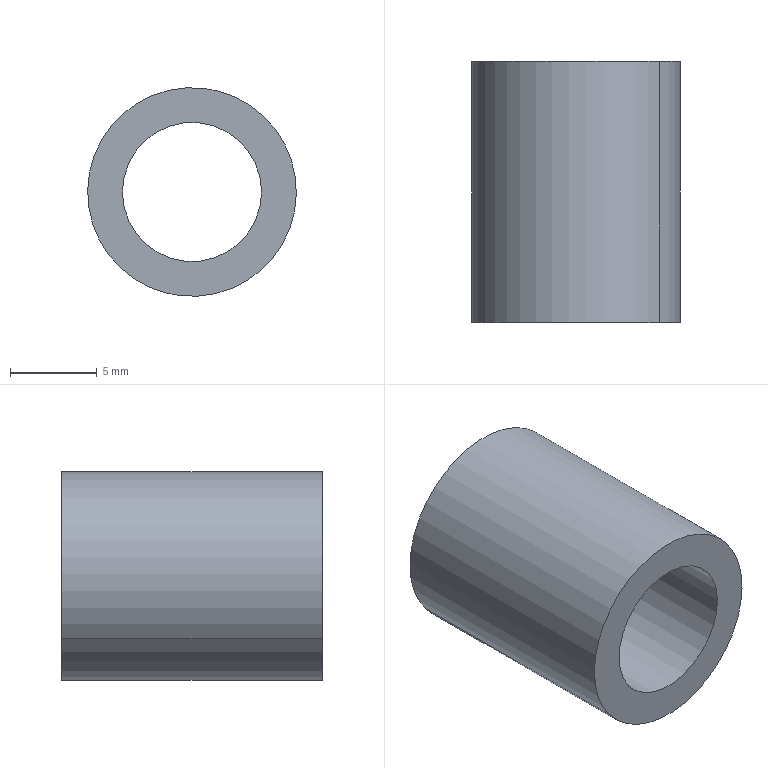Component | SolidWorks | ElectricalBoxAssembly2-1_CopperSleeve10-14-1 | 1 solid | 6 faces | box 12 x 15 x 12 mm | volume 942 mm3 | cylinder 4 | plane 2 | commonest cylinder face diameters 8 x2 12 x2
build123d program:
from build123d import *

# Parameters (mm, degrees)
SKETCH1_R           = 6
SKETCH1_R_2         = 4
BOSS_EXTRUDE1_DEPTH = 7.5


with BuildPart() as part:
    # Sketch1 → Boss-Extrude1 (new, symmetric)
    with BuildSketch(Plane.XY):
        Circle(SKETCH1_R)
        Circle(SKETCH1_R_2, mode=Mode.SUBTRACT)
    extrude(amount=BOSS_EXTRUDE1_DEPTH, both=True)


solid = part.part

# Placed as in the assembly
solid = solid.moved(Location((710.468, 447.166, 1506.399), (90, 0, 0)))
STEP:
#1=CARTESIAN_POINT('',(28.097,17.31,59.402));
#2=VERTEX_POINT('',#1);
#3=CARTESIAN_POINT('',(27.845,17.31,59.212));
#4=VERTEX_POINT('',#3);
#5=CARTESIAN_POINT('',(27.971,17.31,59.307));
#6=DIRECTION('',(-0.,-1.,0.));
#7=DIRECTION('',(-0.7996,0.,-0.6005));
#8=AXIS2_PLACEMENT_3D('',#5,#6,#7);
#9=CIRCLE('',#8,0.1575);
#10=EDGE_CURVE('',#2,#4,#9,.T.);
#11=ORIENTED_EDGE('',*,*,#10,.T.);
#12=CARTESIAN_POINT('',(27.845,17.9,59.212));
#13=VERTEX_POINT('',#12);
#14=CARTESIAN_POINT('',(27.845,17.31,59.212));
#15=DIRECTION('',(0.,1.,-0.));
#16=VECTOR('',#15,39.37);
#17=LINE('',#14,#16);
#18=EDGE_CURVE('',#4,#13,#17,.T.);
#19=ORIENTED_EDGE('',*,*,#18,.T.);
#20=CARTESIAN_POINT('',(28.097,17.9,59.402));
#21=VERTEX_POINT('',#20);
#22=CARTESIAN_POINT('',(27.971,17.9,59.307));
#23=DIRECTION('',(-0.,-1.,0.));
#24=DIRECTION('',(-0.7996,0.,-0.6005));
#25=AXIS2_PLACEMENT_3D('',#22,#23,#24);
#26=CIRCLE('',#25,0.1575);
#27=EDGE_CURVE('',#21,#13,#26,.T.);
#28=ORIENTED_EDGE('',*,*,#27,.F.);
#29=CARTESIAN_POINT('',(28.097,17.31,59.402));
#30=DIRECTION('',(0.,1.,-0.));
#31=VECTOR('',#30,39.37);
#32=LINE('',#29,#31);
#33=EDGE_CURVE('',#2,#21,#32,.T.);
#34=ORIENTED_EDGE('',*,*,#33,.F.);
#35=EDGE_LOOP('',(#11,#19,#28,#34));
#36=FACE_OUTER_BOUND('',#35,.T.);
#37=CARTESIAN_POINT('',(27.971,17.31,59.307));
#38=DIRECTION('',(0.,1.,-0.));
#39=DIRECTION('',(0.7996,0.,0.6005));
#40=AXIS2_PLACEMENT_3D('',#37,#38,#39);
#41=CYLINDRICAL_SURFACE('',#40,0.1575);
#42=ADVANCED_FACE('',(#36),#41,.F.);
#43=CARTESIAN_POINT('',(27.782,17.31,59.165));
#44=VERTEX_POINT('',#43);
#45=CARTESIAN_POINT('',(28.16,17.31,59.449));
#46=VERTEX_POINT('',#45);
#47=CARTESIAN_POINT('',(27.971,17.31,59.307));
#48=DIRECTION('',(-0.,-1.,0.));
#49=DIRECTION('',(-0.7996,0.,-0.6005));
#50=AXIS2_PLACEMENT_3D('',#47,#48,#49);
#51=CIRCLE('',#50,0.2362);
#52=EDGE_CURVE('',#44,#46,#51,.T.);
#53=ORIENTED_EDGE('',*,*,#52,.F.);
#54=CARTESIAN_POINT('',(27.782,17.9,59.165));
#55=VERTEX_POINT('',#54);
#56=CARTESIAN_POINT('',(27.782,17.31,59.165));
#57=DIRECTION('',(0.,1.,-0.));
#58=VECTOR('',#57,39.37);
#59=LINE('',#56,#58);
#60=EDGE_CURVE('',#44,#55,#59,.T.);
#61=ORIENTED_EDGE('',*,*,#60,.T.);
#62=CARTESIAN_POINT('',(28.16,17.9,59.449));
#63=VERTEX_POINT('',#62);
#64=CARTESIAN_POINT('',(27.971,17.9,59.307));
#65=DIRECTION('',(-0.,-1.,0.));
#66=DIRECTION('',(-0.7996,0.,-0.6005));
#67=AXIS2_PLACEMENT_3D('',#64,#65,#66);
#68=CIRCLE('',#67,0.2362);
#69=EDGE_CURVE('',#55,#63,#68,.T.);
#70=ORIENTED_EDGE('',*,*,#69,.T.);
#71=CARTESIAN_POINT('',(28.16,17.31,59.449));
#72=DIRECTION('',(0.,1.,-0.));
#73=VECTOR('',#72,39.37);
#74=LINE('',#71,#73);
#75=EDGE_CURVE('',#46,#63,#74,.T.);
#76=ORIENTED_EDGE('',*,*,#75,.F.);
#77=EDGE_LOOP('',(#53,#61,#70,#76));
#78=FACE_OUTER_BOUND('',#77,.T.);
#79=CARTESIAN_POINT('',(27.971,17.31,59.307));
#80=DIRECTION('',(0.,1.,-0.));
#81=DIRECTION('',(0.7996,0.,0.6005));
#82=AXIS2_PLACEMENT_3D('',#79,#80,#81);
#83=CYLINDRICAL_SURFACE('',#82,0.2362);
#84=ADVANCED_FACE('',(#78),#83,.T.);
#85=CARTESIAN_POINT('',(27.971,17.31,59.307));
#86=DIRECTION('',(-0.,-1.,0.));
#87=DIRECTION('',(-0.7996,0.,-0.6005));
#88=AXIS2_PLACEMENT_3D('',#85,#86,#87);
#89=CIRCLE('',#88,0.2362);
#90=EDGE_CURVE('',#46,#44,#89,.T.);
#91=ORIENTED_EDGE('',*,*,#90,.T.);
#92=ORIENTED_EDGE('',*,*,#52,.T.);
#93=EDGE_LOOP('',(#91,#92));
#94=FACE_OUTER_BOUND('',#93,.T.);
#95=ORIENTED_EDGE('',*,*,#10,.F.);
#96=CARTESIAN_POINT('',(27.971,17.31,59.307));
#97=DIRECTION('',(-0.,-1.,0.));
#98=DIRECTION('',(-0.7996,0.,-0.6005));
#99=AXIS2_PLACEMENT_3D('',#96,#97,#98);
#100=CIRCLE('',#99,0.1575);
#101=EDGE_CURVE('',#4,#2,#100,.T.);
#102=ORIENTED_EDGE('',*,*,#101,.F.);
#103=EDGE_LOOP('',(#95,#102));
#104=FACE_BOUND('',#103,.T.);
#105=CARTESIAN_POINT('',(27.971,17.31,59.307));
#106=DIRECTION('',(-0.,-1.,0.));
#107=DIRECTION('',(-0.7996,-0.,-0.6005));
#108=AXIS2_PLACEMENT_3D('',#105,#106,#107);
#109=PLANE('',#108);
#110=ADVANCED_FACE('',(#94,#104),#109,.T.);
#111=CARTESIAN_POINT('',(27.971,17.9,59.307));
#112=DIRECTION('',(-0.,-1.,0.));
#113=DIRECTION('',(-0.7996,0.,-0.6005));
#114=AXIS2_PLACEMENT_3D('',#111,#112,#113);
#115=CIRCLE('',#114,0.2362);
#116=EDGE_CURVE('',#63,#55,#115,.T.);
#117=ORIENTED_EDGE('',*,*,#116,.F.);
#118=ORIENTED_EDGE('',*,*,#69,.F.);
#119=EDGE_LOOP('',(#117,#118));
#120=FACE_OUTER_BOUND('',#119,.T.);
#121=ORIENTED_EDGE('',*,*,#27,.T.);
#122=CARTESIAN_POINT('',(27.971,17.9,59.307));
#123=DIRECTION('',(-0.,-1.,0.));
#124=DIRECTION('',(-0.7996,0.,-0.6005));
#125=AXIS2_PLACEMENT_3D('',#122,#123,#124);
#126=CIRCLE('',#125,0.1575);
#127=EDGE_CURVE('',#13,#21,#126,.T.);
#128=ORIENTED_EDGE('',*,*,#127,.T.);
#129=EDGE_LOOP('',(#121,#128));
#130=FACE_BOUND('',#129,.T.);
#131=CARTESIAN_POINT('',(27.971,17.9,59.307));
#132=DIRECTION('',(-0.,-1.,0.));
#133=DIRECTION('',(-0.7996,-0.,-0.6005));
#134=AXIS2_PLACEMENT_3D('',#131,#132,#133);
#135=PLANE('',#134);
#136=ADVANCED_FACE('',(#120,#130),#135,.F.);
#137=ORIENTED_EDGE('',*,*,#60,.F.);
#138=ORIENTED_EDGE('',*,*,#90,.F.);
#139=ORIENTED_EDGE('',*,*,#75,.T.);
#140=ORIENTED_EDGE('',*,*,#116,.T.);
#141=EDGE_LOOP('',(#137,#138,#139,#140));
#142=FACE_OUTER_BOUND('',#141,.T.);
#143=CARTESIAN_POINT('',(27.971,17.31,59.307));
#144=DIRECTION('',(0.,1.,-0.));
#145=DIRECTION('',(0.7996,0.,0.6005));
#146=AXIS2_PLACEMENT_3D('',#143,#144,#145);
#147=CYLINDRICAL_SURFACE('',#146,0.2362);
#148=ADVANCED_FACE('',(#142),#147,.T.);
#149=ORIENTED_EDGE('',*,*,#18,.F.);
#150=ORIENTED_EDGE('',*,*,#101,.T.);
#151=ORIENTED_EDGE('',*,*,#33,.T.);
#152=ORIENTED_EDGE('',*,*,#127,.F.);
#153=EDGE_LOOP('',(#149,#150,#151,#152));
#154=FACE_OUTER_BOUND('',#153,.T.);
#155=CARTESIAN_POINT('',(27.971,17.31,59.307));
#156=DIRECTION('',(0.,1.,-0.));
#157=DIRECTION('',(0.7996,0.,0.6005));
#158=AXIS2_PLACEMENT_3D('',#155,#156,#157);
#159=CYLINDRICAL_SURFACE('',#158,0.1575);
#160=ADVANCED_FACE('',(#154),#159,.F.);
#161=CLOSED_SHELL('',(#42,#84,#110,#136,#148,#160));
#162=MANIFOLD_SOLID_BREP('',#161);
#163=CARTESIAN_POINT('',(0.,0.,0.));
#164=DIRECTION('',(0.,0.,1.));
#165=DIRECTION('',(1.,0.,0.));
#166=AXIS2_PLACEMENT_3D('',#163,#164,#165);
#167=(LENGTH_UNIT()NAMED_UNIT(*)SI_UNIT($,.METRE.));
#168=LENGTH_MEASURE_WITH_UNIT(LENGTH_MEASURE(0.0254),#167);
#169=DIMENSIONAL_EXPONENTS(1.,0.,0.,0.,0.,0.,0.);
#170=(CONVERSION_BASED_UNIT('',#168)LENGTH_UNIT()NAMED_UNIT(#169));
#171=UNCERTAINTY_MEASURE_WITH_UNIT(LENGTH_MEASURE(0.00001),#170,'','');
#172=(NAMED_UNIT(*)PLANE_ANGLE_UNIT()SI_UNIT($,.RADIAN.));
#173=(NAMED_UNIT(*)SI_UNIT($,.STERADIAN.)SOLID_ANGLE_UNIT());
#174=(GEOMETRIC_REPRESENTATION_CONTEXT(3)GLOBAL_UNCERTAINTY_ASSIGNED_CONTEXT((#171))GLOBAL_UNIT_ASSIGNED_CONTEXT((#170,#172,#173))REPRESENTATION_CONTEXT('',''));
#175=ADVANCED_BREP_SHAPE_REPRESENTATION('',(#162,#166),#174);
#176=COLOUR_RGB('',0.7922,0.8196,0.9333);
#177=FILL_AREA_STYLE_COLOUR('',#176);
#178=FILL_AREA_STYLE('',(#177));
#179=SURFACE_STYLE_FILL_AREA(#178);
#180=SURFACE_SIDE_STYLE('',(#179));
#181=SURFACE_STYLE_USAGE(.BOTH.,#180);
#182=PRESENTATION_STYLE_ASSIGNMENT((#181));
#183=STYLED_ITEM('',(#182),#162);
#184=(LENGTH_UNIT()NAMED_UNIT(*)SI_UNIT($,.METRE.));
#185=LENGTH_MEASURE_WITH_UNIT(LENGTH_MEASURE(0.0254),#184);
#186=DIMENSIONAL_EXPONENTS(1.,0.,0.,0.,0.,0.,0.);
#187=(CONVERSION_BASED_UNIT('',#185)LENGTH_UNIT()NAMED_UNIT(#186));
#188=UNCERTAINTY_MEASURE_WITH_UNIT(LENGTH_MEASURE(0.00001),#187,'','');
#189=(NAMED_UNIT(*)PLANE_ANGLE_UNIT()SI_UNIT($,.RADIAN.));
#190=(NAMED_UNIT(*)SI_UNIT($,.STERADIAN.)SOLID_ANGLE_UNIT());
#191=(GEOMETRIC_REPRESENTATION_CONTEXT(3)GLOBAL_UNCERTAINTY_ASSIGNED_CONTEXT((#188))GLOBAL_UNIT_ASSIGNED_CONTEXT((#187,#189,#190))REPRESENTATION_CONTEXT('',''));
#192=MECHANICAL_DESIGN_GEOMETRIC_PRESENTATION_REPRESENTATION('',(#183),#191);
#193=PRESENTATION_LAYER_ASSIGNMENT('','',(#183));